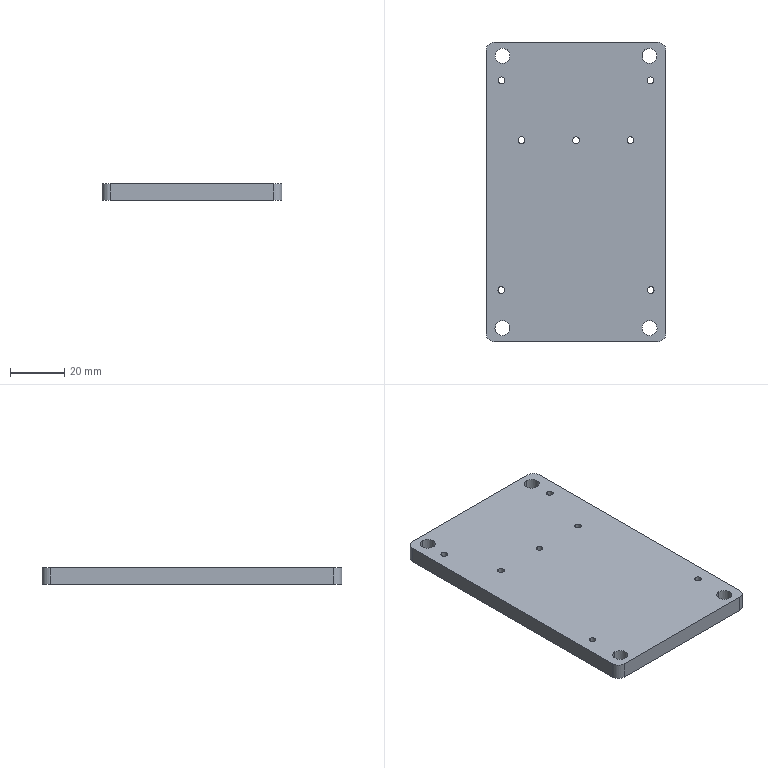CAM job | Mastercam | mm | 8 operations | part box 66 x 110 x 6
1. Facing | 20 - 63 平铣刀
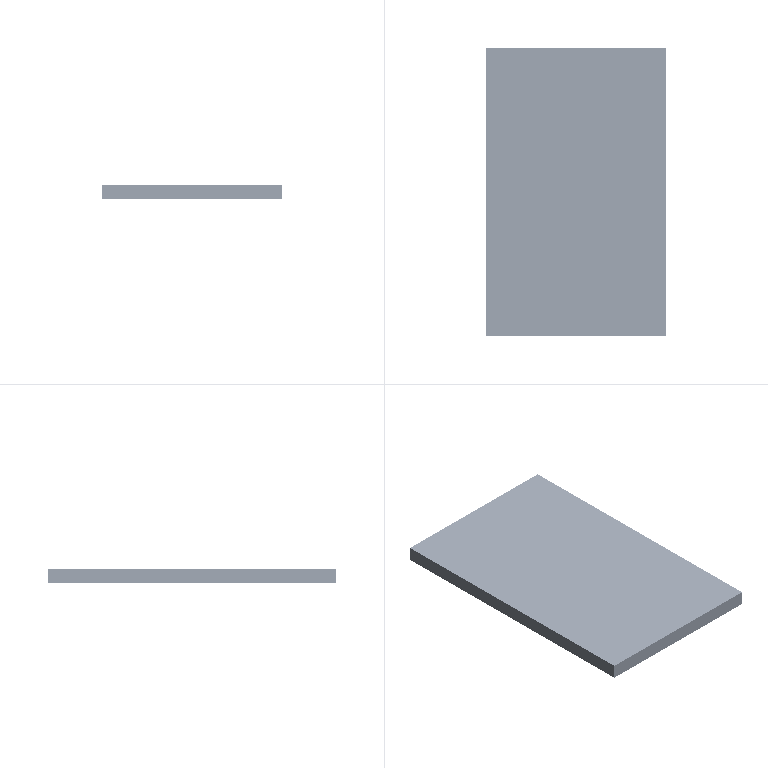2. Contour (Ramp) | 10 - 10 平铣刀
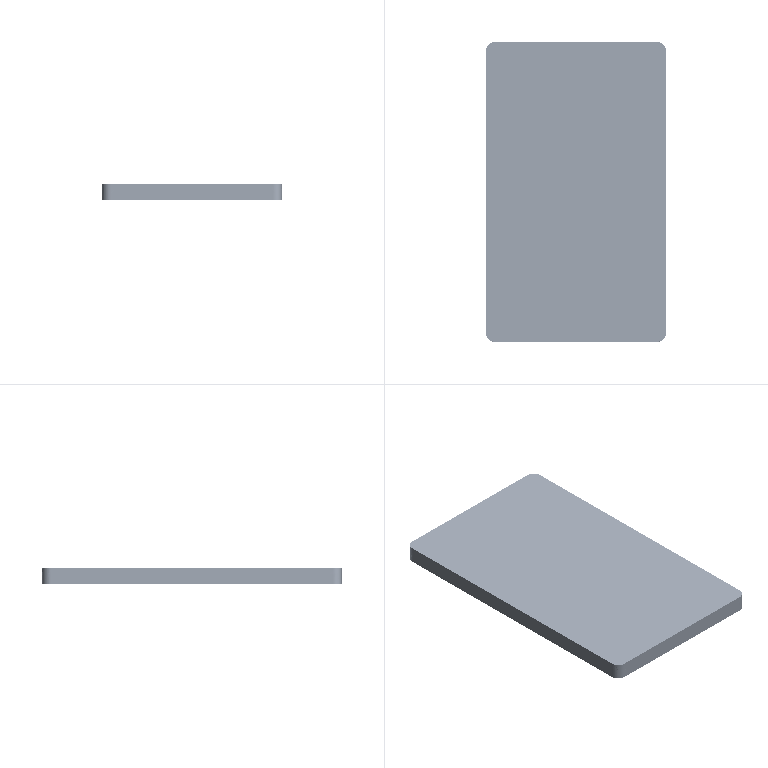3. Contour (2D) | 10 - 10 平铣刀
4. Drill/Counterbore | 7 - 4 倒角刀
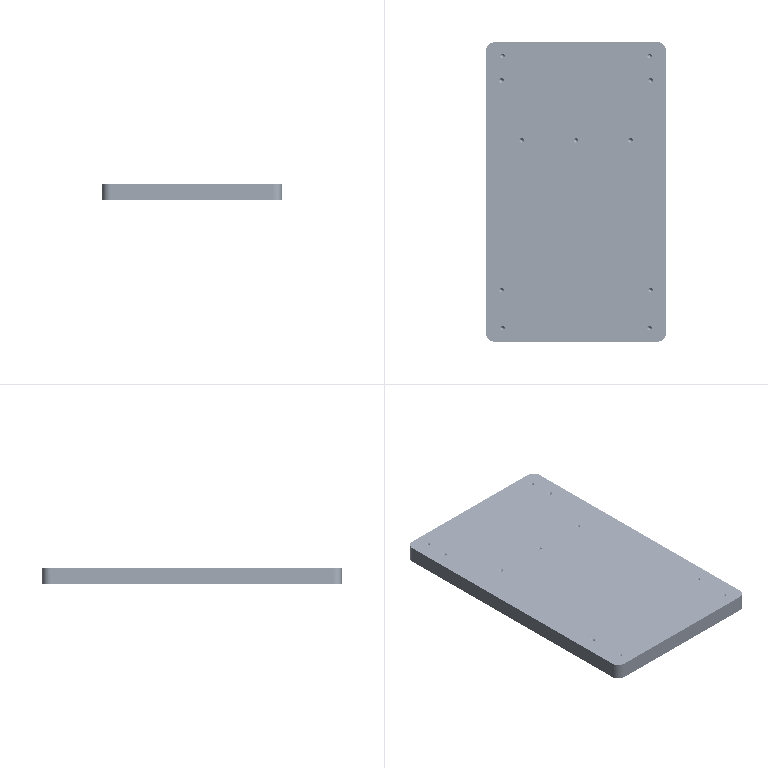5. Contour (2D chamfer) | 7 - 4 倒角刀
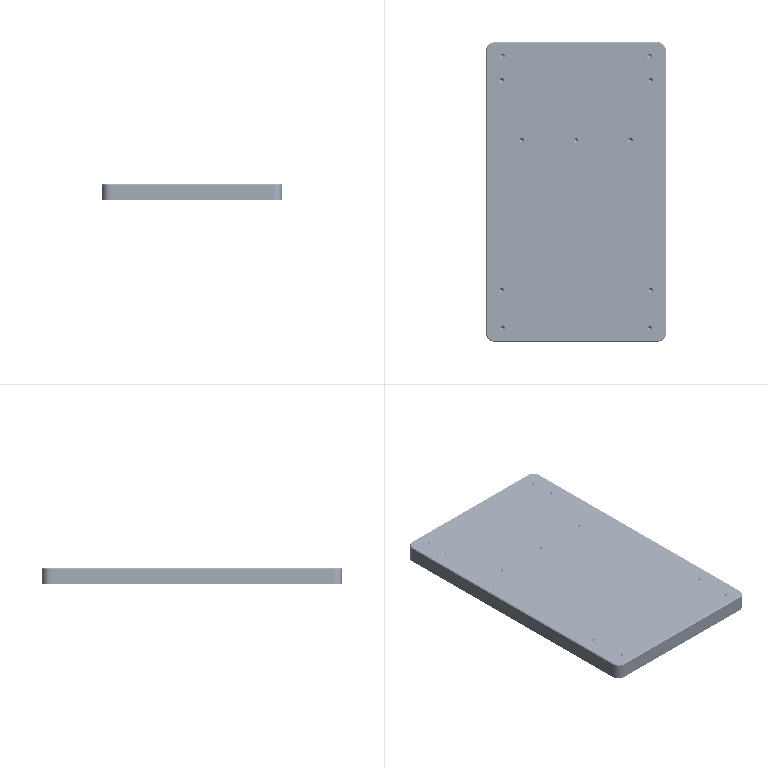6. Facing | 10 - 10 平铣刀
7. Facing | 20 - 63 平铣刀
8. Contour (2D chamfer) | 7 - 4 倒角刀